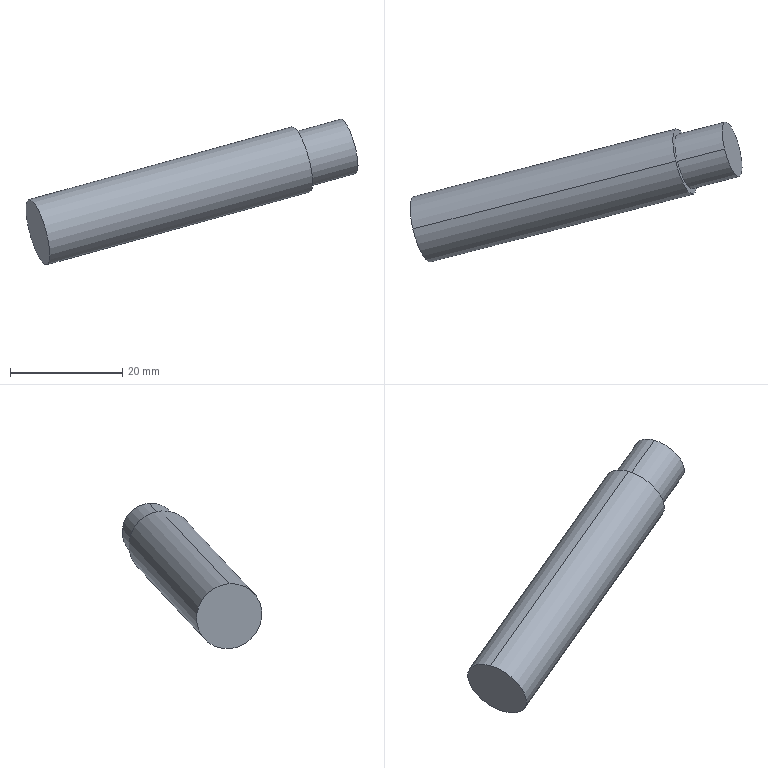Component | SolidWorks | HandleRod10InMulti-HandleNut-2 | 1 solid | 7 faces | box 59.08 x 24.89 x 25.9 mm | volume 6362 mm3 | cylinder 4 | plane 3 | commonest cylinder face diameters 12 x2 10 x2
build123d program:
from build123d import *

# Parameters (mm, degrees)
SKETCH1_R           = 5
BASE_EXTRUDE_DEPTH  = 9
SKETCH2_R           = 6
BOSS_EXTRUDE1_DEPTH = 50


with BuildPart() as part:
    # Sketch1 → Base-Extrude (new body)
    with BuildSketch(Plane.XY):
        Circle(SKETCH1_R)
    extrude(amount=-BASE_EXTRUDE_DEPTH)

    # Sketch2 → Boss-Extrude1 (add)
    with BuildSketch(Plane(origin=(0, 0, -9), x_dir=(-1, 0, 0), z_dir=(0, 0, -1))):
        Circle(SKETCH2_R)
    extrude(amount=BOSS_EXTRUDE1_DEPTH)


solid = part.part

# Placed as in the assembly
solid = solid.moved(Location((17.734, 55.275, -117.569), (-42.94, 69.296, 23.331)))
STEP:
#1=CARTESIAN_POINT('',(-1.538,1.618,-5.002));
#2=VERTEX_POINT('',#1);
#3=CARTESIAN_POINT('',(-1.411,1.615,-5.457));
#4=VERTEX_POINT('',#3);
#5=CARTESIAN_POINT('',(-1.475,1.617,-5.23));
#6=DIRECTION('',(-0.9354,-0.2408,-0.2588));
#7=DIRECTION('',(-0.2682,0.006542,0.9633));
#8=AXIS2_PLACEMENT_3D('',#5,#6,#7);
#9=CIRCLE('',#8,0.2362);
#10=EDGE_CURVE('',#2,#4,#9,.T.);
#11=ORIENTED_EDGE('',*,*,#10,.F.);
#12=CARTESIAN_POINT('',(0.3034,2.092,-4.493));
#13=VERTEX_POINT('',#12);
#14=CARTESIAN_POINT('',(-1.538,1.618,-5.002));
#15=DIRECTION('',(0.9354,0.2408,0.2588));
#16=VECTOR('',#15,39.37);
#17=LINE('',#14,#16);
#18=EDGE_CURVE('',#2,#13,#17,.T.);
#19=ORIENTED_EDGE('',*,*,#18,.T.);
#20=CARTESIAN_POINT('',(0.4301,2.089,-4.948));
#21=VERTEX_POINT('',#20);
#22=CARTESIAN_POINT('',(0.3667,2.091,-4.72));
#23=DIRECTION('',(-0.9354,-0.2408,-0.2588));
#24=DIRECTION('',(-0.2682,0.006542,0.9633));
#25=AXIS2_PLACEMENT_3D('',#22,#23,#24);
#26=CIRCLE('',#25,0.2362);
#27=EDGE_CURVE('',#13,#21,#26,.T.);
#28=ORIENTED_EDGE('',*,*,#27,.T.);
#29=CARTESIAN_POINT('',(-1.411,1.615,-5.457));
#30=DIRECTION('',(0.9354,0.2408,0.2588));
#31=VECTOR('',#30,39.37);
#32=LINE('',#29,#31);
#33=EDGE_CURVE('',#4,#21,#32,.T.);
#34=ORIENTED_EDGE('',*,*,#33,.F.);
#35=EDGE_LOOP('',(#11,#19,#28,#34));
#36=FACE_OUTER_BOUND('',#35,.T.);
#37=CARTESIAN_POINT('',(-1.475,1.617,-5.23));
#38=DIRECTION('',(0.9354,0.2408,0.2588));
#39=DIRECTION('',(0.2682,-0.006542,-0.9633));
#40=AXIS2_PLACEMENT_3D('',#37,#38,#39);
#41=CYLINDRICAL_SURFACE('',#40,0.2362);
#42=ADVANCED_FACE('',(#36),#41,.T.);
#43=CARTESIAN_POINT('',(0.4195,2.09,-4.91));
#44=VERTEX_POINT('',#43);
#45=CARTESIAN_POINT('',(0.3139,2.092,-4.531));
#46=VERTEX_POINT('',#45);
#47=CARTESIAN_POINT('',(0.3667,2.091,-4.72));
#48=DIRECTION('',(0.9354,0.2408,0.2588));
#49=DIRECTION('',(-0.2682,0.006542,0.9633));
#50=AXIS2_PLACEMENT_3D('',#47,#48,#49);
#51=CIRCLE('',#50,0.1969);
#52=EDGE_CURVE('',#44,#46,#51,.T.);
#53=ORIENTED_EDGE('',*,*,#52,.T.);
#54=CARTESIAN_POINT('',(0.6454,2.177,-4.439));
#55=VERTEX_POINT('',#54);
#56=CARTESIAN_POINT('',(0.3139,2.092,-4.531));
#57=DIRECTION('',(0.9354,0.2408,0.2588));
#58=VECTOR('',#57,39.37);
#59=LINE('',#56,#58);
#60=EDGE_CURVE('',#46,#55,#59,.T.);
#61=ORIENTED_EDGE('',*,*,#60,.T.);
#62=CARTESIAN_POINT('',(0.751,2.175,-4.818));
#63=VERTEX_POINT('',#62);
#64=CARTESIAN_POINT('',(0.6982,2.176,-4.629));
#65=DIRECTION('',(0.9354,0.2408,0.2588));
#66=DIRECTION('',(0.2682,-0.006542,-0.9633));
#67=AXIS2_PLACEMENT_3D('',#64,#65,#66);
#68=CIRCLE('',#67,0.1969);
#69=EDGE_CURVE('',#63,#55,#68,.T.);
#70=ORIENTED_EDGE('',*,*,#69,.F.);
#71=CARTESIAN_POINT('',(0.4195,2.09,-4.91));
#72=DIRECTION('',(0.9354,0.2408,0.2588));
#73=VECTOR('',#72,39.37);
#74=LINE('',#71,#73);
#75=EDGE_CURVE('',#44,#63,#74,.T.);
#76=ORIENTED_EDGE('',*,*,#75,.F.);
#77=EDGE_LOOP('',(#53,#61,#70,#76));
#78=FACE_OUTER_BOUND('',#77,.T.);
#79=CARTESIAN_POINT('',(0.3667,2.091,-4.72));
#80=DIRECTION('',(0.9354,0.2408,0.2588));
#81=DIRECTION('',(0.2682,-0.006542,-0.9633));
#82=AXIS2_PLACEMENT_3D('',#79,#80,#81);
#83=CYLINDRICAL_SURFACE('',#82,0.1969);
#84=ADVANCED_FACE('',(#78),#83,.T.);
#85=ORIENTED_EDGE('',*,*,#60,.F.);
#86=CARTESIAN_POINT('',(0.3667,2.091,-4.72));
#87=DIRECTION('',(0.9354,0.2408,0.2588));
#88=DIRECTION('',(-0.2682,0.006542,0.9633));
#89=AXIS2_PLACEMENT_3D('',#86,#87,#88);
#90=CIRCLE('',#89,0.1969);
#91=EDGE_CURVE('',#46,#44,#90,.T.);
#92=ORIENTED_EDGE('',*,*,#91,.T.);
#93=ORIENTED_EDGE('',*,*,#75,.T.);
#94=CARTESIAN_POINT('',(0.6982,2.176,-4.629));
#95=DIRECTION('',(0.9354,0.2408,0.2588));
#96=DIRECTION('',(0.2682,-0.006542,-0.9633));
#97=AXIS2_PLACEMENT_3D('',#94,#95,#96);
#98=CIRCLE('',#97,0.1969);
#99=EDGE_CURVE('',#55,#63,#98,.T.);
#100=ORIENTED_EDGE('',*,*,#99,.F.);
#101=EDGE_LOOP('',(#85,#92,#93,#100));
#102=FACE_OUTER_BOUND('',#101,.T.);
#103=CARTESIAN_POINT('',(0.3667,2.091,-4.72));
#104=DIRECTION('',(0.9354,0.2408,0.2588));
#105=DIRECTION('',(0.2682,-0.006542,-0.9633));
#106=AXIS2_PLACEMENT_3D('',#103,#104,#105);
#107=CYLINDRICAL_SURFACE('',#106,0.1969);
#108=ADVANCED_FACE('',(#102),#107,.T.);
#109=ORIENTED_EDGE('',*,*,#69,.T.);
#110=ORIENTED_EDGE('',*,*,#99,.T.);
#111=EDGE_LOOP('',(#109,#110));
#112=FACE_OUTER_BOUND('',#111,.T.);
#113=CARTESIAN_POINT('',(0.6982,2.176,-4.629));
#114=DIRECTION('',(0.9354,0.2408,0.2588));
#115=DIRECTION('',(0.2682,-0.006542,-0.9633));
#116=AXIS2_PLACEMENT_3D('',#113,#114,#115);
#117=PLANE('',#116);
#118=ADVANCED_FACE('',(#112),#117,.T.);
#119=ORIENTED_EDGE('',*,*,#18,.F.);
#120=CARTESIAN_POINT('',(-1.475,1.617,-5.23));
#121=DIRECTION('',(-0.9354,-0.2408,-0.2588));
#122=DIRECTION('',(-0.2682,0.006542,0.9633));
#123=AXIS2_PLACEMENT_3D('',#120,#121,#122);
#124=CIRCLE('',#123,0.2362);
#125=EDGE_CURVE('',#4,#2,#124,.T.);
#126=ORIENTED_EDGE('',*,*,#125,.F.);
#127=ORIENTED_EDGE('',*,*,#33,.T.);
#128=CARTESIAN_POINT('',(0.3667,2.091,-4.72));
#129=DIRECTION('',(-0.9354,-0.2408,-0.2588));
#130=DIRECTION('',(-0.2682,0.006542,0.9633));
#131=AXIS2_PLACEMENT_3D('',#128,#129,#130);
#132=CIRCLE('',#131,0.2362);
#133=EDGE_CURVE('',#21,#13,#132,.T.);
#134=ORIENTED_EDGE('',*,*,#133,.T.);
#135=EDGE_LOOP('',(#119,#126,#127,#134));
#136=FACE_OUTER_BOUND('',#135,.T.);
#137=CARTESIAN_POINT('',(-1.475,1.617,-5.23));
#138=DIRECTION('',(0.9354,0.2408,0.2588));
#139=DIRECTION('',(0.2682,-0.006542,-0.9633));
#140=AXIS2_PLACEMENT_3D('',#137,#138,#139);
#141=CYLINDRICAL_SURFACE('',#140,0.2362);
#142=ADVANCED_FACE('',(#136),#141,.T.);
#143=ORIENTED_EDGE('',*,*,#125,.T.);
#144=ORIENTED_EDGE('',*,*,#10,.T.);
#145=EDGE_LOOP('',(#143,#144));
#146=FACE_OUTER_BOUND('',#145,.T.);
#147=CARTESIAN_POINT('',(-1.475,1.617,-5.23));
#148=DIRECTION('',(-0.9354,-0.2408,-0.2588));
#149=DIRECTION('',(-0.2682,0.006542,0.9633));
#150=AXIS2_PLACEMENT_3D('',#147,#148,#149);
#151=PLANE('',#150);
#152=ADVANCED_FACE('',(#146),#151,.T.);
#153=ORIENTED_EDGE('',*,*,#52,.F.);
#154=ORIENTED_EDGE('',*,*,#91,.F.);
#155=EDGE_LOOP('',(#153,#154));
#156=FACE_BOUND('',#155,.T.);
#157=ORIENTED_EDGE('',*,*,#133,.F.);
#158=ORIENTED_EDGE('',*,*,#27,.F.);
#159=EDGE_LOOP('',(#157,#158));
#160=FACE_OUTER_BOUND('',#159,.T.);
#161=CARTESIAN_POINT('',(0.3667,2.091,-4.72));
#162=DIRECTION('',(-0.9354,-0.2408,-0.2588));
#163=DIRECTION('',(-0.2682,0.006542,0.9633));
#164=AXIS2_PLACEMENT_3D('',#161,#162,#163);
#165=PLANE('',#164);
#166=ADVANCED_FACE('',(#156,#160),#165,.F.);
#167=CLOSED_SHELL('',(#42,#84,#108,#118,#142,#152,#166));
#168=MANIFOLD_SOLID_BREP('',#167);
#169=CARTESIAN_POINT('',(0.,0.,0.));
#170=DIRECTION('',(0.,0.,1.));
#171=DIRECTION('',(1.,0.,0.));
#172=AXIS2_PLACEMENT_3D('',#169,#170,#171);
#173=(LENGTH_UNIT()NAMED_UNIT(*)SI_UNIT($,.METRE.));
#174=LENGTH_MEASURE_WITH_UNIT(LENGTH_MEASURE(0.0254),#173);
#175=DIMENSIONAL_EXPONENTS(1.,0.,0.,0.,0.,0.,0.);
#176=(CONVERSION_BASED_UNIT('',#174)LENGTH_UNIT()NAMED_UNIT(#175));
#177=UNCERTAINTY_MEASURE_WITH_UNIT(LENGTH_MEASURE(0.00001),#176,'','');
#178=(NAMED_UNIT(*)PLANE_ANGLE_UNIT()SI_UNIT($,.RADIAN.));
#179=(NAMED_UNIT(*)SI_UNIT($,.STERADIAN.)SOLID_ANGLE_UNIT());
#180=(GEOMETRIC_REPRESENTATION_CONTEXT(3)GLOBAL_UNCERTAINTY_ASSIGNED_CONTEXT((#177))GLOBAL_UNIT_ASSIGNED_CONTEXT((#176,#178,#179))REPRESENTATION_CONTEXT('',''));
#181=ADVANCED_BREP_SHAPE_REPRESENTATION('',(#168,#172),#180);
#182=COLOUR_RGB('',0.7922,0.8196,0.9333);
#183=FILL_AREA_STYLE_COLOUR('',#182);
#184=FILL_AREA_STYLE('',(#183));
#185=SURFACE_STYLE_FILL_AREA(#184);
#186=SURFACE_SIDE_STYLE('',(#185));
#187=SURFACE_STYLE_USAGE(.BOTH.,#186);
#188=PRESENTATION_STYLE_ASSIGNMENT((#187));
#189=STYLED_ITEM('',(#188),#168);
#190=(LENGTH_UNIT()NAMED_UNIT(*)SI_UNIT($,.METRE.));
#191=LENGTH_MEASURE_WITH_UNIT(LENGTH_MEASURE(0.0254),#190);
#192=DIMENSIONAL_EXPONENTS(1.,0.,0.,0.,0.,0.,0.);
#193=(CONVERSION_BASED_UNIT('',#191)LENGTH_UNIT()NAMED_UNIT(#192));
#194=UNCERTAINTY_MEASURE_WITH_UNIT(LENGTH_MEASURE(0.00001),#193,'','');
#195=(NAMED_UNIT(*)PLANE_ANGLE_UNIT()SI_UNIT($,.RADIAN.));
#196=(NAMED_UNIT(*)SI_UNIT($,.STERADIAN.)SOLID_ANGLE_UNIT());
#197=(GEOMETRIC_REPRESENTATION_CONTEXT(3)GLOBAL_UNCERTAINTY_ASSIGNED_CONTEXT((#194))GLOBAL_UNIT_ASSIGNED_CONTEXT((#193,#195,#196))REPRESENTATION_CONTEXT('',''));
#198=MECHANICAL_DESIGN_GEOMETRIC_PRESENTATION_REPRESENTATION('',(#189),#197);
#199=PRESENTATION_LAYER_ASSIGNMENT('','',(#189));